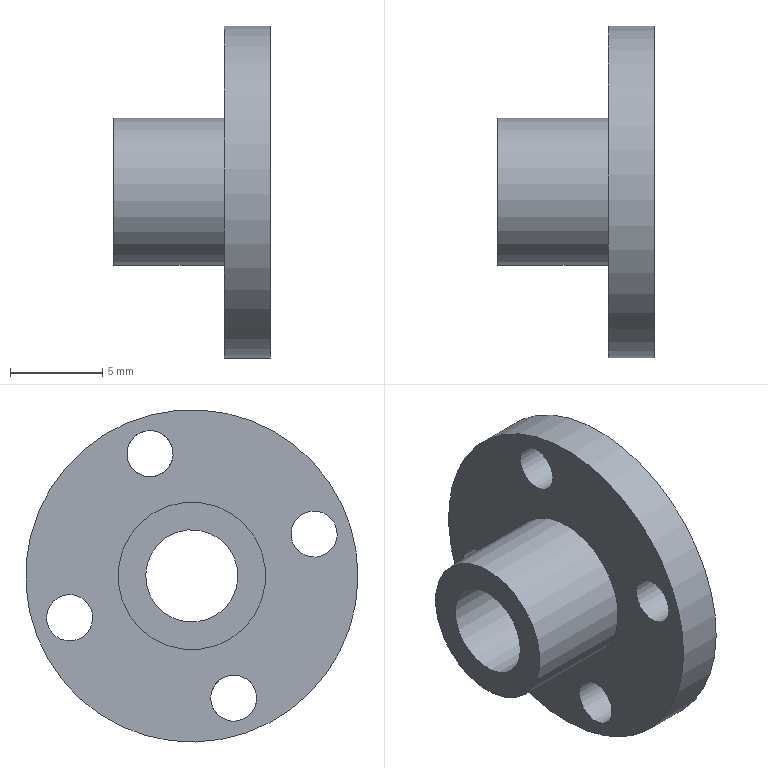Component | NX | END_CAP_3_OUTER_CAP | 1 solid | 10 faces | volume 722 mm3 | cylinder 7 | plane 3 | commonest cylinder face diameters 2.5 x4 8 x1 18 x1 5 x1